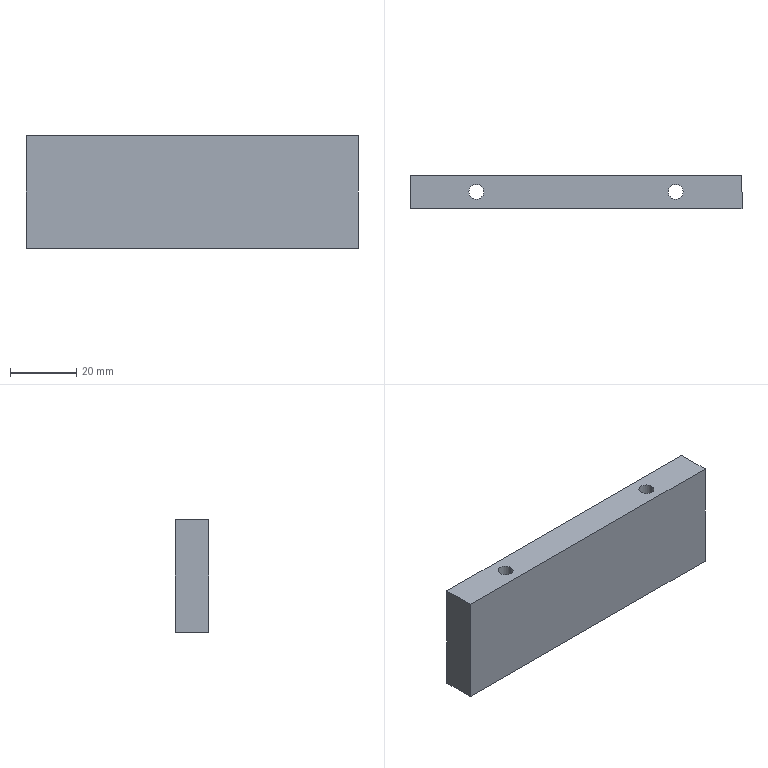Component | SolidWorks | 07-1111-1 | 1 solid | 28 faces | box 100 x 10 x 34 mm | volume 30538 mm3 | cylinder 14 | plane 8 | cone 6 | commonest cylinder face diameters 3.3 x6 8 x4 4.5 x4 | material AL6061(GB)Natural Anodized
build123d program:
from build123d import *

# Parameters (mm, degrees)
SKETCH1_W                                       = 100
SKETCH1_H                                       = 10
EXTRUDE1_DEPTH                                  = 34
M4_HEX_SOCKET_HEAD_CAP_SCREW_CBORE1_D           = 4.5
M4_HEX_SOCKET_HEAD_CAP_SCREW_CBORE1_CBORE_D     = 8
M4_HEX_SOCKET_HEAD_CAP_SCREW_CBORE1_CBORE_DEPTH = 30
M4_TAPPED_HOLE1_D                               = 3.3
M4_TAPPED_HOLE1_DEPTH                           = 12.1
M4_TAPPED_HOLE1_TIP                             = 0.9914


with BuildPart() as part:
    # Sketch1 → Extrude1 (new body)
    with BuildSketch(Plane.XY):
        with Locations((50, 5)):
            Rectangle(SKETCH1_W, SKETCH1_H)
    extrude(amount=EXTRUDE1_DEPTH)

    # M4 Hex Socket Head Cap Screw CBORE1 (through all)
    with Locations(Plane.XY.offset(34)):
        with Locations((20, 5), (80, 5)):
            CounterBoreHole(M4_HEX_SOCKET_HEAD_CAP_SCREW_CBORE1_D / 2, M4_HEX_SOCKET_HEAD_CAP_SCREW_CBORE1_CBORE_D / 2, M4_HEX_SOCKET_HEAD_CAP_SCREW_CBORE1_CBORE_DEPTH)

    # M4 Tapped Hole1
    with Locations(Plane.XY.offset(34)):
        with Locations((8, 5), (50, 5), (92, 5)):
            Hole(M4_TAPPED_HOLE1_D / 2, depth=M4_TAPPED_HOLE1_DEPTH)
            with Locations((0, 0, -(M4_TAPPED_HOLE1_DEPTH + M4_TAPPED_HOLE1_TIP / 2))):  # 118° drill point
                Cone(0, M4_TAPPED_HOLE1_D / 2, M4_TAPPED_HOLE1_TIP, mode=Mode.SUBTRACT)


solid = part.part

# Placed as in the assembly
solid = solid.moved(Location((-64.57, 60, -32), (180, 0, 0)))
STEP:
#1=CARTESIAN_POINT('',(-2.292,2.165,-2.122));
#2=VERTEX_POINT('',#1);
#3=CARTESIAN_POINT('',(-2.162,2.165,-2.122));
#4=VERTEX_POINT('',#3);
#5=CARTESIAN_POINT('',(-2.227,2.165,-2.122));
#6=DIRECTION('',(0.,0.,-1.));
#7=DIRECTION('',(1.,0.,0.));
#8=AXIS2_PLACEMENT_3D('',#5,#6,#7);
#9=CIRCLE('',#8,0.06496);
#10=EDGE_CURVE('',#2,#4,#9,.T.);
#11=ORIENTED_EDGE('',*,*,#10,.F.);
#12=CARTESIAN_POINT('',(-2.292,2.165,-2.598));
#13=VERTEX_POINT('',#12);
#14=CARTESIAN_POINT('',(-2.292,2.165,-2.598));
#15=DIRECTION('',(0.,0.,-1.));
#16=VECTOR('',#15,39.37);
#17=LINE('',#14,#16);
#18=EDGE_CURVE('',#2,#13,#17,.T.);
#19=ORIENTED_EDGE('',*,*,#18,.T.);
#20=CARTESIAN_POINT('',(-2.162,2.165,-2.598));
#21=VERTEX_POINT('',#20);
#22=CARTESIAN_POINT('',(-2.227,2.165,-2.598));
#23=DIRECTION('',(0.,0.,-1.));
#24=DIRECTION('',(1.,0.,0.));
#25=AXIS2_PLACEMENT_3D('',#22,#23,#24);
#26=CIRCLE('',#25,0.06496);
#27=EDGE_CURVE('',#13,#21,#26,.T.);
#28=ORIENTED_EDGE('',*,*,#27,.T.);
#29=CARTESIAN_POINT('',(-2.162,2.165,-2.598));
#30=DIRECTION('',(0.,0.,-1.));
#31=VECTOR('',#30,39.37);
#32=LINE('',#29,#31);
#33=EDGE_CURVE('',#4,#21,#32,.T.);
#34=ORIENTED_EDGE('',*,*,#33,.F.);
#35=EDGE_LOOP('',(#11,#19,#28,#34));
#36=FACE_OUTER_BOUND('',#35,.T.);
#37=CARTESIAN_POINT('',(-2.227,2.165,-2.598));
#38=DIRECTION('',(0.,0.,-1.));
#39=DIRECTION('',(1.,0.,0.));
#40=AXIS2_PLACEMENT_3D('',#37,#38,#39);
#41=CYLINDRICAL_SURFACE('',#40,0.06496);
#42=ADVANCED_FACE('',(#36),#41,.F.);
#43=CARTESIAN_POINT('',(-2.227,2.165,-2.083));
#44=VERTEX_POINT('',#43);
#45=CARTESIAN_POINT('',(-2.162,2.165,-2.122));
#46=DIRECTION('',(0.8572,0.,-0.515));
#47=VECTOR('',#46,39.37);
#48=LINE('',#45,#47);
#49=EDGE_CURVE('',#44,#4,#48,.T.);
#50=ORIENTED_EDGE('',*,*,#49,.F.);
#51=CARTESIAN_POINT('',(-2.292,2.165,-2.122));
#52=DIRECTION('',(-0.8572,-0.,-0.515));
#53=VECTOR('',#52,39.37);
#54=LINE('',#51,#53);
#55=EDGE_CURVE('',#44,#2,#54,.T.);
#56=ORIENTED_EDGE('',*,*,#55,.T.);
#57=ORIENTED_EDGE('',*,*,#10,.T.);
#58=EDGE_LOOP('',(#50,#56,#57));
#59=FACE_OUTER_BOUND('',#58,.T.);
#60=CARTESIAN_POINT('',(-2.227,2.165,-2.122));
#61=DIRECTION('',(0.,0.,-1.));
#62=DIRECTION('',(1.,0.,0.));
#63=AXIS2_PLACEMENT_3D('',#60,#61,#62);
#64=CONICAL_SURFACE('',#63,0.06496,1.03);
#65=ADVANCED_FACE('',(#59),#64,.F.);
#66=CARTESIAN_POINT('',(-0.6386,2.165,-2.122));
#67=VERTEX_POINT('',#66);
#68=CARTESIAN_POINT('',(-0.5087,2.165,-2.122));
#69=VERTEX_POINT('',#68);
#70=CARTESIAN_POINT('',(-0.5736,2.165,-2.122));
#71=DIRECTION('',(0.,0.,-1.));
#72=DIRECTION('',(1.,0.,0.));
#73=AXIS2_PLACEMENT_3D('',#70,#71,#72);
#74=CIRCLE('',#73,0.06496);
#75=EDGE_CURVE('',#67,#69,#74,.T.);
#76=ORIENTED_EDGE('',*,*,#75,.F.);
#77=CARTESIAN_POINT('',(-0.6386,2.165,-2.598));
#78=VERTEX_POINT('',#77);
#79=CARTESIAN_POINT('',(-0.6386,2.165,-2.598));
#80=DIRECTION('',(0.,0.,-1.));
#81=VECTOR('',#80,39.37);
#82=LINE('',#79,#81);
#83=EDGE_CURVE('',#67,#78,#82,.T.);
#84=ORIENTED_EDGE('',*,*,#83,.T.);
#85=CARTESIAN_POINT('',(-0.5087,2.165,-2.598));
#86=VERTEX_POINT('',#85);
#87=CARTESIAN_POINT('',(-0.5736,2.165,-2.598));
#88=DIRECTION('',(0.,0.,-1.));
#89=DIRECTION('',(1.,0.,0.));
#90=AXIS2_PLACEMENT_3D('',#87,#88,#89);
#91=CIRCLE('',#90,0.06496);
#92=EDGE_CURVE('',#78,#86,#91,.T.);
#93=ORIENTED_EDGE('',*,*,#92,.T.);
#94=CARTESIAN_POINT('',(-0.5087,2.165,-2.598));
#95=DIRECTION('',(0.,0.,-1.));
#96=VECTOR('',#95,39.37);
#97=LINE('',#94,#96);
#98=EDGE_CURVE('',#69,#86,#97,.T.);
#99=ORIENTED_EDGE('',*,*,#98,.F.);
#100=EDGE_LOOP('',(#76,#84,#93,#99));
#101=FACE_OUTER_BOUND('',#100,.T.);
#102=CARTESIAN_POINT('',(-0.5736,2.165,-2.598));
#103=DIRECTION('',(0.,0.,-1.));
#104=DIRECTION('',(1.,0.,0.));
#105=AXIS2_PLACEMENT_3D('',#102,#103,#104);
#106=CYLINDRICAL_SURFACE('',#105,0.06496);
#107=ADVANCED_FACE('',(#101),#106,.F.);
#108=CARTESIAN_POINT('',(-0.5736,2.165,-2.083));
#109=VERTEX_POINT('',#108);
#110=CARTESIAN_POINT('',(-0.5087,2.165,-2.122));
#111=DIRECTION('',(0.8572,0.,-0.515));
#112=VECTOR('',#111,39.37);
#113=LINE('',#110,#112);
#114=EDGE_CURVE('',#109,#69,#113,.T.);
#115=ORIENTED_EDGE('',*,*,#114,.F.);
#116=CARTESIAN_POINT('',(-0.6386,2.165,-2.122));
#117=DIRECTION('',(-0.8572,-0.,-0.515));
#118=VECTOR('',#117,39.37);
#119=LINE('',#116,#118);
#120=EDGE_CURVE('',#109,#67,#119,.T.);
#121=ORIENTED_EDGE('',*,*,#120,.T.);
#122=ORIENTED_EDGE('',*,*,#75,.T.);
#123=EDGE_LOOP('',(#115,#121,#122));
#124=FACE_OUTER_BOUND('',#123,.T.);
#125=CARTESIAN_POINT('',(-0.5736,2.165,-2.122));
#126=DIRECTION('',(0.,0.,-1.));
#127=DIRECTION('',(1.,0.,0.));
#128=AXIS2_PLACEMENT_3D('',#125,#126,#127);
#129=CONICAL_SURFACE('',#128,0.06496,1.03);
#130=ADVANCED_FACE('',(#124),#129,.F.);
#131=CARTESIAN_POINT('',(1.015,2.165,-2.122));
#132=VERTEX_POINT('',#131);
#133=CARTESIAN_POINT('',(1.145,2.165,-2.122));
#134=VERTEX_POINT('',#133);
#135=CARTESIAN_POINT('',(1.08,2.165,-2.122));
#136=DIRECTION('',(0.,0.,-1.));
#137=DIRECTION('',(1.,0.,0.));
#138=AXIS2_PLACEMENT_3D('',#135,#136,#137);
#139=CIRCLE('',#138,0.06496);
#140=EDGE_CURVE('',#132,#134,#139,.T.);
#141=ORIENTED_EDGE('',*,*,#140,.F.);
#142=CARTESIAN_POINT('',(1.015,2.165,-2.598));
#143=VERTEX_POINT('',#142);
#144=CARTESIAN_POINT('',(1.015,2.165,-2.598));
#145=DIRECTION('',(0.,0.,-1.));
#146=VECTOR('',#145,39.37);
#147=LINE('',#144,#146);
#148=EDGE_CURVE('',#132,#143,#147,.T.);
#149=ORIENTED_EDGE('',*,*,#148,.T.);
#150=CARTESIAN_POINT('',(1.145,2.165,-2.598));
#151=VERTEX_POINT('',#150);
#152=CARTESIAN_POINT('',(1.08,2.165,-2.598));
#153=DIRECTION('',(0.,0.,-1.));
#154=DIRECTION('',(1.,0.,0.));
#155=AXIS2_PLACEMENT_3D('',#152,#153,#154);
#156=CIRCLE('',#155,0.06496);
#157=EDGE_CURVE('',#143,#151,#156,.T.);
#158=ORIENTED_EDGE('',*,*,#157,.T.);
#159=CARTESIAN_POINT('',(1.145,2.165,-2.598));
#160=DIRECTION('',(0.,0.,-1.));
#161=VECTOR('',#160,39.37);
#162=LINE('',#159,#161);
#163=EDGE_CURVE('',#134,#151,#162,.T.);
#164=ORIENTED_EDGE('',*,*,#163,.F.);
#165=EDGE_LOOP('',(#141,#149,#158,#164));
#166=FACE_OUTER_BOUND('',#165,.T.);
#167=CARTESIAN_POINT('',(1.08,2.165,-2.598));
#168=DIRECTION('',(0.,0.,-1.));
#169=DIRECTION('',(1.,0.,0.));
#170=AXIS2_PLACEMENT_3D('',#167,#168,#169);
#171=CYLINDRICAL_SURFACE('',#170,0.06496);
#172=ADVANCED_FACE('',(#166),#171,.F.);
#173=CARTESIAN_POINT('',(1.08,2.165,-2.083));
#174=VERTEX_POINT('',#173);
#175=CARTESIAN_POINT('',(1.145,2.165,-2.122));
#176=DIRECTION('',(0.8572,0.,-0.515));
#177=VECTOR('',#176,39.37);
#178=LINE('',#175,#177);
#179=EDGE_CURVE('',#174,#134,#178,.T.);
#180=ORIENTED_EDGE('',*,*,#179,.F.);
#181=CARTESIAN_POINT('',(1.015,2.165,-2.122));
#182=DIRECTION('',(-0.8572,-0.,-0.515));
#183=VECTOR('',#182,39.37);
#184=LINE('',#181,#183);
#185=EDGE_CURVE('',#174,#132,#184,.T.);
#186=ORIENTED_EDGE('',*,*,#185,.T.);
#187=ORIENTED_EDGE('',*,*,#140,.T.);
#188=EDGE_LOOP('',(#180,#186,#187));
#189=FACE_OUTER_BOUND('',#188,.T.);
#190=CARTESIAN_POINT('',(1.08,2.165,-2.122));
#191=DIRECTION('',(0.,0.,-1.));
#192=DIRECTION('',(1.,0.,0.));
#193=AXIS2_PLACEMENT_3D('',#190,#191,#192);
#194=CONICAL_SURFACE('',#193,0.06496,1.03);
#195=ADVANCED_FACE('',(#189),#194,.F.);
#196=CARTESIAN_POINT('',(-1.912,2.165,-1.417));
#197=VERTEX_POINT('',#196);
#198=CARTESIAN_POINT('',(-1.597,2.165,-1.417));
#199=VERTEX_POINT('',#198);
#200=CARTESIAN_POINT('',(-1.755,2.165,-1.417));
#201=DIRECTION('',(0.,0.,-1.));
#202=DIRECTION('',(1.,0.,0.));
#203=AXIS2_PLACEMENT_3D('',#200,#201,#202);
#204=CIRCLE('',#203,0.1575);
#205=EDGE_CURVE('',#197,#199,#204,.T.);
#206=ORIENTED_EDGE('',*,*,#205,.F.);
#207=CARTESIAN_POINT('',(-1.912,2.165,-2.598));
#208=VERTEX_POINT('',#207);
#209=CARTESIAN_POINT('',(-1.912,2.165,-2.598));
#210=DIRECTION('',(0.,0.,-1.));
#211=VECTOR('',#210,39.37);
#212=LINE('',#209,#211);
#213=EDGE_CURVE('',#197,#208,#212,.T.);
#214=ORIENTED_EDGE('',*,*,#213,.T.);
#215=CARTESIAN_POINT('',(-1.597,2.165,-2.598));
#216=VERTEX_POINT('',#215);
#217=CARTESIAN_POINT('',(-1.755,2.165,-2.598));
#218=DIRECTION('',(0.,0.,-1.));
#219=DIRECTION('',(1.,0.,0.));
#220=AXIS2_PLACEMENT_3D('',#217,#218,#219);
#221=CIRCLE('',#220,0.1575);
#222=EDGE_CURVE('',#208,#216,#221,.T.);
#223=ORIENTED_EDGE('',*,*,#222,.T.);
#224=CARTESIAN_POINT('',(-1.597,2.165,-2.598));
#225=DIRECTION('',(0.,0.,-1.));
#226=VECTOR('',#225,39.37);
#227=LINE('',#224,#226);
#228=EDGE_CURVE('',#199,#216,#227,.T.);
#229=ORIENTED_EDGE('',*,*,#228,.F.);
#230=EDGE_LOOP('',(#206,#214,#223,#229));
#231=FACE_OUTER_BOUND('',#230,.T.);
#232=CARTESIAN_POINT('',(-1.755,2.165,-2.598));
#233=DIRECTION('',(0.,0.,-1.));
#234=DIRECTION('',(1.,0.,0.));
#235=AXIS2_PLACEMENT_3D('',#232,#233,#234);
#236=CYLINDRICAL_SURFACE('',#235,0.1575);
#237=ADVANCED_FACE('',(#231),#236,.F.);
#238=CARTESIAN_POINT('',(-1.843,2.165,-1.26));
#239=VERTEX_POINT('',#238);
#240=CARTESIAN_POINT('',(-1.666,2.165,-1.26));
#241=VERTEX_POINT('',#240);
#242=CARTESIAN_POINT('',(-1.755,2.165,-1.26));
#243=DIRECTION('',(0.,0.,-1.));
#244=DIRECTION('',(1.,0.,0.));
#245=AXIS2_PLACEMENT_3D('',#242,#243,#244);
#246=CIRCLE('',#245,0.08858);
#247=EDGE_CURVE('',#239,#241,#246,.T.);
#248=ORIENTED_EDGE('',*,*,#247,.F.);
#249=CARTESIAN_POINT('',(-1.843,2.165,-1.417));
#250=VERTEX_POINT('',#249);
#251=CARTESIAN_POINT('',(-1.843,2.165,-2.598));
#252=DIRECTION('',(0.,0.,-1.));
#253=VECTOR('',#252,39.37);
#254=LINE('',#251,#253);
#255=EDGE_CURVE('',#239,#250,#254,.T.);
#256=ORIENTED_EDGE('',*,*,#255,.T.);
#257=CARTESIAN_POINT('',(-1.666,2.165,-1.417));
#258=VERTEX_POINT('',#257);
#259=CARTESIAN_POINT('',(-1.755,2.165,-1.417));
#260=DIRECTION('',(0.,0.,-1.));
#261=DIRECTION('',(1.,0.,0.));
#262=AXIS2_PLACEMENT_3D('',#259,#260,#261);
#263=CIRCLE('',#262,0.08858);
#264=EDGE_CURVE('',#250,#258,#263,.T.);
#265=ORIENTED_EDGE('',*,*,#264,.T.);
#266=CARTESIAN_POINT('',(-1.666,2.165,-2.598));
#267=DIRECTION('',(0.,0.,-1.));
#268=VECTOR('',#267,39.37);
#269=LINE('',#266,#268);
#270=EDGE_CURVE('',#241,#258,#269,.T.);
#271=ORIENTED_EDGE('',*,*,#270,.F.);
#272=EDGE_LOOP('',(#248,#256,#265,#271));
#273=FACE_OUTER_BOUND('',#272,.T.);
#274=CARTESIAN_POINT('',(-1.755,2.165,-2.598));
#275=DIRECTION('',(0.,0.,-1.));
#276=DIRECTION('',(1.,0.,0.));
#277=AXIS2_PLACEMENT_3D('',#274,#275,#276);
#278=CYLINDRICAL_SURFACE('',#277,0.08858);
#279=ADVANCED_FACE('',(#273),#278,.F.);
#280=CARTESIAN_POINT('',(0.45,2.165,-1.417));
#281=VERTEX_POINT('',#280);
#282=CARTESIAN_POINT('',(0.765,2.165,-1.417));
#283=VERTEX_POINT('',#282);
#284=CARTESIAN_POINT('',(0.6075,2.165,-1.417));
#285=DIRECTION('',(0.,0.,-1.));
#286=DIRECTION('',(1.,0.,0.));
#287=AXIS2_PLACEMENT_3D('',#284,#285,#286);
#288=CIRCLE('',#287,0.1575);
#289=EDGE_CURVE('',#281,#283,#288,.T.);
#290=ORIENTED_EDGE('',*,*,#289,.F.);
#291=CARTESIAN_POINT('',(0.45,2.165,-2.598));
#292=VERTEX_POINT('',#291);
#293=CARTESIAN_POINT('',(0.45,2.165,-2.598));
#294=DIRECTION('',(0.,0.,-1.));
#295=VECTOR('',#294,39.37);
#296=LINE('',#293,#295);
#297=EDGE_CURVE('',#281,#292,#296,.T.);
#298=ORIENTED_EDGE('',*,*,#297,.T.);
#299=CARTESIAN_POINT('',(0.765,2.165,-2.598));
#300=VERTEX_POINT('',#299);
#301=CARTESIAN_POINT('',(0.6075,2.165,-2.598));
#302=DIRECTION('',(0.,0.,-1.));
#303=DIRECTION('',(1.,0.,0.));
#304=AXIS2_PLACEMENT_3D('',#301,#302,#303);
#305=CIRCLE('',#304,0.1575);
#306=EDGE_CURVE('',#292,#300,#305,.T.);
#307=ORIENTED_EDGE('',*,*,#306,.T.);
#308=CARTESIAN_POINT('',(0.765,2.165,-2.598));
#309=DIRECTION('',(0.,0.,-1.));
#310=VECTOR('',#309,39.37);
#311=LINE('',#308,#310);
#312=EDGE_CURVE('',#283,#300,#311,.T.);
#313=ORIENTED_EDGE('',*,*,#312,.F.);
#314=EDGE_LOOP('',(#290,#298,#307,#313));
#315=FACE_OUTER_BOUND('',#314,.T.);
#316=CARTESIAN_POINT('',(0.6075,2.165,-2.598));
#317=DIRECTION('',(0.,0.,-1.));
#318=DIRECTION('',(1.,0.,0.));
#319=AXIS2_PLACEMENT_3D('',#316,#317,#318);
#320=CYLINDRICAL_SURFACE('',#319,0.1575);
#321=ADVANCED_FACE('',(#315),#320,.F.);
#322=CARTESIAN_POINT('',(0.5189,2.165,-1.26));
#323=VERTEX_POINT('',#322);
#324=CARTESIAN_POINT('',(0.6961,2.165,-1.26));
#325=VERTEX_POINT('',#324);
#326=CARTESIAN_POINT('',(0.6075,2.165,-1.26));
#327=DIRECTION('',(0.,0.,-1.));
#328=DIRECTION('',(1.,0.,0.));
#329=AXIS2_PLACEMENT_3D('',#326,#327,#328);
#330=CIRCLE('',#329,0.08858);
#331=EDGE_CURVE('',#323,#325,#330,.T.);
#332=ORIENTED_EDGE('',*,*,#331,.F.);
#333=CARTESIAN_POINT('',(0.5189,2.165,-1.417));
#334=VERTEX_POINT('',#333);
#335=CARTESIAN_POINT('',(0.5189,2.165,-2.598));
#336=DIRECTION('',(0.,0.,-1.));
#337=VECTOR('',#336,39.37);
#338=LINE('',#335,#337);
#339=EDGE_CURVE('',#323,#334,#338,.T.);
#340=ORIENTED_EDGE('',*,*,#339,.T.);
#341=CARTESIAN_POINT('',(0.6961,2.165,-1.417));
#342=VERTEX_POINT('',#341);
#343=CARTESIAN_POINT('',(0.6075,2.165,-1.417));
#344=DIRECTION('',(0.,0.,-1.));
#345=DIRECTION('',(1.,0.,0.));
#346=AXIS2_PLACEMENT_3D('',#343,#344,#345);
#347=CIRCLE('',#346,0.08858);
#348=EDGE_CURVE('',#334,#342,#347,.T.);
#349=ORIENTED_EDGE('',*,*,#348,.T.);
#350=CARTESIAN_POINT('',(0.6961,2.165,-2.598));
#351=DIRECTION('',(0.,0.,-1.));
#352=VECTOR('',#351,39.37);
#353=LINE('',#350,#352);
#354=EDGE_CURVE('',#325,#342,#353,.T.);
#355=ORIENTED_EDGE('',*,*,#354,.F.);
#356=EDGE_LOOP('',(#332,#340,#349,#355));
#357=FACE_OUTER_BOUND('',#356,.T.);
#358=CARTESIAN_POINT('',(0.6075,2.165,-2.598));
#359=DIRECTION('',(0.,0.,-1.));
#360=DIRECTION('',(1.,0.,0.));
#361=AXIS2_PLACEMENT_3D('',#358,#359,#360);
#362=CYLINDRICAL_SURFACE('',#361,0.08858);
#363=ADVANCED_FACE('',(#357),#362,.F.);
#364=CARTESIAN_POINT('',(-2.542,1.969,-1.26));
#365=VERTEX_POINT('',#364);
#366=CARTESIAN_POINT('',(-2.542,2.362,-1.26));
#367=VERTEX_POINT('',#366);
#368=CARTESIAN_POINT('',(-2.542,2.362,-1.26));
#369=DIRECTION('',(-0.,1.,-0.));
#370=VECTOR('',#369,39.37);
#371=LINE('',#368,#370);
#372=EDGE_CURVE('',#365,#367,#371,.T.);
#373=ORIENTED_EDGE('',*,*,#372,.T.);
#374=CARTESIAN_POINT('',(-2.542,2.362,-2.598));
#375=VERTEX_POINT('',#374);
#376=CARTESIAN_POINT('',(-2.542,2.362,-2.598));
#377=DIRECTION('',(-0.,-0.,1.));
#378=VECTOR('',#377,39.37);
#379=LINE('',#376,#378);
#380=EDGE_CURVE('',#375,#367,#379,.T.);
#381=ORIENTED_EDGE('',*,*,#380,.F.);
#382=CARTESIAN_POINT('',(-2.542,1.969,-2.598));
#383=VERTEX_POINT('',#382);
#384=CARTESIAN_POINT('',(-2.542,2.362,-2.598));
#385=DIRECTION('',(-0.,1.,-0.));
#386=VECTOR('',#385,39.37);
#387=LINE('',#384,#386);
#388=EDGE_CURVE('',#383,#375,#387,.T.);
#389=ORIENTED_EDGE('',*,*,#388,.F.);
#390=CARTESIAN_POINT('',(-2.542,1.969,-2.598));
#391=DIRECTION('',(-0.,-0.,1.));
#392=VECTOR('',#391,39.37);
#393=LINE('',#390,#392);
#394=EDGE_CURVE('',#383,#365,#393,.T.);
#395=ORIENTED_EDGE('',*,*,#394,.T.);
#396=EDGE_LOOP('',(#373,#381,#389,#395));
#397=FACE_OUTER_BOUND('',#396,.T.);
#398=CARTESIAN_POINT('',(-2.542,2.362,-2.598));
#399=DIRECTION('',(1.,0.,0.));
#400=DIRECTION('',(-0.,-0.,1.));
#401=AXIS2_PLACEMENT_3D('',#398,#399,#400);
#402=PLANE('',#401);
#403=ADVANCED_FACE('',(#397),#402,.F.);
#404=CARTESIAN_POINT('',(1.395,2.362,-1.26));
#405=VERTEX_POINT('',#404);
#406=CARTESIAN_POINT('',(-2.542,2.362,-1.26));
#407=DIRECTION('',(1.,0.,0.));
#408=VECTOR('',#407,39.37);
#409=LINE('',#406,#408);
#410=EDGE_CURVE('',#367,#405,#409,.T.);
#411=ORIENTED_EDGE('',*,*,#410,.T.);
#412=CARTESIAN_POINT('',(1.395,2.362,-2.598));
#413=VERTEX_POINT('',#412);
#414=CARTESIAN_POINT('',(1.395,2.362,-2.598));
#415=DIRECTION('',(-0.,-0.,1.));
#416=VECTOR('',#415,39.37);
#417=LINE('',#414,#416);
#418=EDGE_CURVE('',#413,#405,#417,.T.);
#419=ORIENTED_EDGE('',*,*,#418,.F.);
#420=CARTESIAN_POINT('',(-2.542,2.362,-2.598));
#421=DIRECTION('',(1.,0.,0.));
#422=VECTOR('',#421,39.37);
#423=LINE('',#420,#422);
#424=EDGE_CURVE('',#375,#413,#423,.T.);
#425=ORIENTED_EDGE('',*,*,#424,.F.);
#426=ORIENTED_EDGE('',*,*,#380,.T.);
#427=EDGE_LOOP('',(#411,#419,#425,#426));
#428=FACE_OUTER_BOUND('',#427,.T.);
#429=CARTESIAN_POINT('',(-2.542,2.362,-2.598));
#430=DIRECTION('',(0.,-1.,-0.));
#431=DIRECTION('',(0.,0.,-1.));
#432=AXIS2_PLACEMENT_3D('',#429,#430,#431);
#433=PLANE('',#432);
#434=ADVANCED_FACE('',(#428),#433,.F.);
#435=CARTESIAN_POINT('',(1.395,1.969,-1.26));
#436=VERTEX_POINT('',#435);
#437=CARTESIAN_POINT('',(1.395,2.362,-1.26));
#438=DIRECTION('',(0.,-1.,0.));
#439=VECTOR('',#438,39.37);
#440=LINE('',#437,#439);
#441=EDGE_CURVE('',#405,#436,#440,.T.);
#442=ORIENTED_EDGE('',*,*,#441,.T.);
#443=CARTESIAN_POINT('',(1.395,1.969,-2.598));
#444=VERTEX_POINT('',#443);
#445=CARTESIAN_POINT('',(1.395,1.969,-2.598));
#446=DIRECTION('',(-0.,-0.,1.));
#447=VECTOR('',#446,39.37);
#448=LINE('',#445,#447);
#449=EDGE_CURVE('',#444,#436,#448,.T.);
#450=ORIENTED_EDGE('',*,*,#449,.F.);
#451=CARTESIAN_POINT('',(1.395,2.362,-2.598));
#452=DIRECTION('',(0.,-1.,0.));
#453=VECTOR('',#452,39.37);
#454=LINE('',#451,#453);
#455=EDGE_CURVE('',#413,#444,#454,.T.);
#456=ORIENTED_EDGE('',*,*,#455,.F.);
#457=ORIENTED_EDGE('',*,*,#418,.T.);
#458=EDGE_LOOP('',(#442,#450,#456,#457));
#459=FACE_OUTER_BOUND('',#458,.T.);
#460=CARTESIAN_POINT('',(1.395,2.362,-2.598));
#461=DIRECTION('',(-1.,-0.,-0.));
#462=DIRECTION('',(0.,0.,-1.));
#463=AXIS2_PLACEMENT_3D('',#460,#461,#462);
#464=PLANE('',#463);
#465=ADVANCED_FACE('',(#459),#464,.F.);
#466=CARTESIAN_POINT('',(-2.542,1.969,-1.26));
#467=DIRECTION('',(-1.,-0.,-0.));
#468=VECTOR('',#467,39.37);
#469=LINE('',#466,#468);
#470=EDGE_CURVE('',#436,#365,#469,.T.);
#471=ORIENTED_EDGE('',*,*,#470,.T.);
#472=ORIENTED_EDGE('',*,*,#394,.F.);
#473=CARTESIAN_POINT('',(-2.542,1.969,-2.598));
#474=DIRECTION('',(-1.,-0.,-0.));
#475=VECTOR('',#474,39.37);
#476=LINE('',#473,#475);
#477=EDGE_CURVE('',#444,#383,#476,.T.);
#478=ORIENTED_EDGE('',*,*,#477,.F.);
#479=ORIENTED_EDGE('',*,*,#449,.T.);
#480=EDGE_LOOP('',(#471,#472,#478,#479));
#481=FACE_OUTER_BOUND('',#480,.T.);
#482=CARTESIAN_POINT('',(-2.542,1.969,-2.598));
#483=DIRECTION('',(-0.,1.,0.));
#484=DIRECTION('',(-0.,-0.,1.));
#485=AXIS2_PLACEMENT_3D('',#482,#483,#484);
#486=PLANE('',#485);
#487=ADVANCED_FACE('',(#481),#486,.F.);
#488=CARTESIAN_POINT('',(-2.227,2.165,-2.598));
#489=DIRECTION('',(0.,0.,-1.));
#490=DIRECTION('',(1.,0.,0.));
#491=AXIS2_PLACEMENT_3D('',#488,#489,#490);
#492=CIRCLE('',#491,0.06496);
#493=EDGE_CURVE('',#21,#13,#492,.T.);
#494=ORIENTED_EDGE('',*,*,#493,.F.);
#495=ORIENTED_EDGE('',*,*,#27,.F.);
#496=EDGE_LOOP('',(#494,#495));
#497=FACE_BOUND('',#496,.T.);
#498=CARTESIAN_POINT('',(-0.5736,2.165,-2.598));
#499=DIRECTION('',(0.,0.,-1.));
#500=DIRECTION('',(1.,0.,0.));
#501=AXIS2_PLACEMENT_3D('',#498,#499,#500);
#502=CIRCLE('',#501,0.06496);
#503=EDGE_CURVE('',#86,#78,#502,.T.);
#504=ORIENTED_EDGE('',*,*,#503,.F.);
#505=ORIENTED_EDGE('',*,*,#92,.F.);
#506=EDGE_LOOP('',(#504,#505));
#507=FACE_BOUND('',#506,.T.);
#508=CARTESIAN_POINT('',(1.08,2.165,-2.598));
#509=DIRECTION('',(0.,0.,-1.));
#510=DIRECTION('',(1.,0.,0.));
#511=AXIS2_PLACEMENT_3D('',#508,#509,#510);
#512=CIRCLE('',#511,0.06496);
#513=EDGE_CURVE('',#151,#143,#512,.T.);
#514=ORIENTED_EDGE('',*,*,#513,.F.);
#515=ORIENTED_EDGE('',*,*,#157,.F.);
#516=EDGE_LOOP('',(#514,#515));
#517=FACE_BOUND('',#516,.T.);
#518=CARTESIAN_POINT('',(-1.755,2.165,-2.598));
#519=DIRECTION('',(0.,0.,-1.));
#520=DIRECTION('',(1.,0.,0.));
#521=AXIS2_PLACEMENT_3D('',#518,#519,#520);
#522=CIRCLE('',#521,0.1575);
#523=EDGE_CURVE('',#216,#208,#522,.T.);
#524=ORIENTED_EDGE('',*,*,#523,.F.);
#525=ORIENTED_EDGE('',*,*,#222,.F.);
#526=EDGE_LOOP('',(#524,#525));
#527=FACE_BOUND('',#526,.T.);
#528=CARTESIAN_POINT('',(0.6075,2.165,-2.598));
#529=DIRECTION('',(0.,0.,-1.));
#530=DIRECTION('',(1.,0.,0.));
#531=AXIS2_PLACEMENT_3D('',#528,#529,#530);
#532=CIRCLE('',#531,0.1575);
#533=EDGE_CURVE('',#300,#292,#532,.T.);
#534=ORIENTED_EDGE('',*,*,#533,.F.);
#535=ORIENTED_EDGE('',*,*,#306,.F.);
#536=EDGE_LOOP('',(#534,#535));
#537=FACE_BOUND('',#536,.T.);
#538=ORIENTED_EDGE('',*,*,#388,.T.);
#539=ORIENTED_EDGE('',*,*,#424,.T.);
#540=ORIENTED_EDGE('',*,*,#455,.T.);
#541=ORIENTED_EDGE('',*,*,#477,.T.);
#542=EDGE_LOOP('',(#538,#539,#540,#541));
#543=FACE_OUTER_BOUND('',#542,.T.);
#544=CARTESIAN_POINT('',(-2.542,1.969,-2.598));
#545=DIRECTION('',(-0.,-0.,1.));
#546=DIRECTION('',(-1.,-0.,-0.));
#547=AXIS2_PLACEMENT_3D('',#544,#545,#546);
#548=PLANE('',#547);
#549=ADVANCED_FACE('',(#497,#507,#517,#527,#537,#543),#548,.F.);
#550=CARTESIAN_POINT('',(-1.755,2.165,-1.26));
#551=DIRECTION('',(0.,0.,-1.));
#552=DIRECTION('',(1.,0.,0.));
#553=AXIS2_PLACEMENT_3D('',#550,#551,#552);
#554=CIRCLE('',#553,0.08858);
#555=EDGE_CURVE('',#241,#239,#554,.T.);
#556=ORIENTED_EDGE('',*,*,#555,.T.);
#557=ORIENTED_EDGE('',*,*,#247,.T.);
#558=EDGE_LOOP('',(#556,#557));
#559=FACE_BOUND('',#558,.T.);
#560=CARTESIAN_POINT('',(0.6075,2.165,-1.26));
#561=DIRECTION('',(0.,0.,-1.));
#562=DIRECTION('',(1.,0.,0.));
#563=AXIS2_PLACEMENT_3D('',#560,#561,#562);
#564=CIRCLE('',#563,0.08858);
#565=EDGE_CURVE('',#325,#323,#564,.T.);
#566=ORIENTED_EDGE('',*,*,#565,.T.);
#567=ORIENTED_EDGE('',*,*,#331,.T.);
#568=EDGE_LOOP('',(#566,#567));
#569=FACE_BOUND('',#568,.T.);
#570=ORIENTED_EDGE('',*,*,#372,.F.);
#571=ORIENTED_EDGE('',*,*,#470,.F.);
#572=ORIENTED_EDGE('',*,*,#441,.F.);
#573=ORIENTED_EDGE('',*,*,#410,.F.);
#574=EDGE_LOOP('',(#570,#571,#572,#573));
#575=FACE_OUTER_BOUND('',#574,.T.);
#576=CARTESIAN_POINT('',(-2.542,1.969,-1.26));
#577=DIRECTION('',(-0.,-0.,1.));
#578=DIRECTION('',(-1.,-0.,-0.));
#579=AXIS2_PLACEMENT_3D('',#576,#577,#578);
#580=PLANE('',#579);
#581=ADVANCED_FACE('',(#559,#569,#575),#580,.T.);
#582=ORIENTED_EDGE('',*,*,#339,.F.);
#583=ORIENTED_EDGE('',*,*,#565,.F.);
#584=ORIENTED_EDGE('',*,*,#354,.T.);
#585=CARTESIAN_POINT('',(0.6075,2.165,-1.417));
#586=DIRECTION('',(0.,0.,-1.));
#587=DIRECTION('',(1.,0.,0.));
#588=AXIS2_PLACEMENT_3D('',#585,#586,#587);
#589=CIRCLE('',#588,0.08858);
#590=EDGE_CURVE('',#342,#334,#589,.T.);
#591=ORIENTED_EDGE('',*,*,#590,.T.);
#592=EDGE_LOOP('',(#582,#583,#584,#591));
#593=FACE_OUTER_BOUND('',#592,.T.);
#594=CARTESIAN_POINT('',(0.6075,2.165,-2.598));
#595=DIRECTION('',(0.,0.,-1.));
#596=DIRECTION('',(1.,0.,0.));
#597=AXIS2_PLACEMENT_3D('',#594,#595,#596);
#598=CYLINDRICAL_SURFACE('',#597,0.08858);
#599=ADVANCED_FACE('',(#593),#598,.F.);
#600=ORIENTED_EDGE('',*,*,#590,.F.);
#601=ORIENTED_EDGE('',*,*,#348,.F.);
#602=EDGE_LOOP('',(#600,#601));
#603=FACE_BOUND('',#602,.T.);
#604=CARTESIAN_POINT('',(0.6075,2.165,-1.417));
#605=DIRECTION('',(0.,0.,-1.));
#606=DIRECTION('',(1.,0.,0.));
#607=AXIS2_PLACEMENT_3D('',#604,#605,#606);
#608=CIRCLE('',#607,0.1575);
#609=EDGE_CURVE('',#283,#281,#608,.T.);
#610=ORIENTED_EDGE('',*,*,#609,.T.);
#611=ORIENTED_EDGE('',*,*,#289,.T.);
#612=EDGE_LOOP('',(#610,#611));
#613=FACE_OUTER_BOUND('',#612,.T.);
#614=CARTESIAN_POINT('',(0.6961,2.165,-1.417));
#615=DIRECTION('',(-0.,-0.,1.));
#616=DIRECTION('',(-1.,-0.,-0.));
#617=AXIS2_PLACEMENT_3D('',#614,#615,#616);
#618=PLANE('',#617);
#619=ADVANCED_FACE('',(#603,#613),#618,.F.);
#620=ORIENTED_EDGE('',*,*,#297,.F.);
#621=ORIENTED_EDGE('',*,*,#609,.F.);
#622=ORIENTED_EDGE('',*,*,#312,.T.);
#623=ORIENTED_EDGE('',*,*,#533,.T.);
#624=EDGE_LOOP('',(#620,#621,#622,#623));
#625=FACE_OUTER_BOUND('',#624,.T.);
#626=CARTESIAN_POINT('',(0.6075,2.165,-2.598));
#627=DIRECTION('',(0.,0.,-1.));
#628=DIRECTION('',(1.,0.,0.));
#629=AXIS2_PLACEMENT_3D('',#626,#627,#628);
#630=CYLINDRICAL_SURFACE('',#629,0.1575);
#631=ADVANCED_FACE('',(#625),#630,.F.);
#632=ORIENTED_EDGE('',*,*,#255,.F.);
#633=ORIENTED_EDGE('',*,*,#555,.F.);
#634=ORIENTED_EDGE('',*,*,#270,.T.);
#635=CARTESIAN_POINT('',(-1.755,2.165,-1.417));
#636=DIRECTION('',(0.,0.,-1.));
#637=DIRECTION('',(1.,0.,0.));
#638=AXIS2_PLACEMENT_3D('',#635,#636,#637);
#639=CIRCLE('',#638,0.08858);
#640=EDGE_CURVE('',#258,#250,#639,.T.);
#641=ORIENTED_EDGE('',*,*,#640,.T.);
#642=EDGE_LOOP('',(#632,#633,#634,#641));
#643=FACE_OUTER_BOUND('',#642,.T.);
#644=CARTESIAN_POINT('',(-1.755,2.165,-2.598));
#645=DIRECTION('',(0.,0.,-1.));
#646=DIRECTION('',(1.,0.,0.));
#647=AXIS2_PLACEMENT_3D('',#644,#645,#646);
#648=CYLINDRICAL_SURFACE('',#647,0.08858);
#649=ADVANCED_FACE('',(#643),#648,.F.);
#650=ORIENTED_EDGE('',*,*,#640,.F.);
#651=ORIENTED_EDGE('',*,*,#264,.F.);
#652=EDGE_LOOP('',(#650,#651));
#653=FACE_BOUND('',#652,.T.);
#654=CARTESIAN_POINT('',(-1.755,2.165,-1.417));
#655=DIRECTION('',(0.,0.,-1.));
#656=DIRECTION('',(1.,0.,0.));
#657=AXIS2_PLACEMENT_3D('',#654,#655,#656);
#658=CIRCLE('',#657,0.1575);
#659=EDGE_CURVE('',#199,#197,#658,.T.);
#660=ORIENTED_EDGE('',*,*,#659,.T.);
#661=ORIENTED_EDGE('',*,*,#205,.T.);
#662=EDGE_LOOP('',(#660,#661));
#663=FACE_OUTER_BOUND('',#662,.T.);
#664=CARTESIAN_POINT('',(-1.666,2.165,-1.417));
#665=DIRECTION('',(-0.,-0.,1.));
#666=DIRECTION('',(-1.,-0.,-0.));
#667=AXIS2_PLACEMENT_3D('',#664,#665,#666);
#668=PLANE('',#667);
#669=ADVANCED_FACE('',(#653,#663),#668,.F.);
#670=ORIENTED_EDGE('',*,*,#213,.F.);
#671=ORIENTED_EDGE('',*,*,#659,.F.);
#672=ORIENTED_EDGE('',*,*,#228,.T.);
#673=ORIENTED_EDGE('',*,*,#523,.T.);
#674=EDGE_LOOP('',(#670,#671,#672,#673));
#675=FACE_OUTER_BOUND('',#674,.T.);
#676=CARTESIAN_POINT('',(-1.755,2.165,-2.598));
#677=DIRECTION('',(0.,0.,-1.));
#678=DIRECTION('',(1.,0.,0.));
#679=AXIS2_PLACEMENT_3D('',#676,#677,#678);
#680=CYLINDRICAL_SURFACE('',#679,0.1575);
#681=ADVANCED_FACE('',(#675),#680,.F.);
#682=ORIENTED_EDGE('',*,*,#185,.F.);
#683=ORIENTED_EDGE('',*,*,#179,.T.);
#684=CARTESIAN_POINT('',(1.08,2.165,-2.122));
#685=DIRECTION('',(0.,0.,-1.));
#686=DIRECTION('',(1.,0.,0.));
#687=AXIS2_PLACEMENT_3D('',#684,#685,#686);
#688=CIRCLE('',#687,0.06496);
#689=EDGE_CURVE('',#134,#132,#688,.T.);
#690=ORIENTED_EDGE('',*,*,#689,.T.);
#691=EDGE_LOOP('',(#682,#683,#690));
#692=FACE_OUTER_BOUND('',#691,.T.);
#693=CARTESIAN_POINT('',(1.08,2.165,-2.122));
#694=DIRECTION('',(0.,0.,-1.));
#695=DIRECTION('',(1.,0.,0.));
#696=AXIS2_PLACEMENT_3D('',#693,#694,#695);
#697=CONICAL_SURFACE('',#696,0.06496,1.03);
#698=ADVANCED_FACE('',(#692),#697,.F.);
#699=ORIENTED_EDGE('',*,*,#148,.F.);
#700=ORIENTED_EDGE('',*,*,#689,.F.);
#701=ORIENTED_EDGE('',*,*,#163,.T.);
#702=ORIENTED_EDGE('',*,*,#513,.T.);
#703=EDGE_LOOP('',(#699,#700,#701,#702));
#704=FACE_OUTER_BOUND('',#703,.T.);
#705=CARTESIAN_POINT('',(1.08,2.165,-2.598));
#706=DIRECTION('',(0.,0.,-1.));
#707=DIRECTION('',(1.,0.,0.));
#708=AXIS2_PLACEMENT_3D('',#705,#706,#707);
#709=CYLINDRICAL_SURFACE('',#708,0.06496);
#710=ADVANCED_FACE('',(#704),#709,.F.);
#711=ORIENTED_EDGE('',*,*,#120,.F.);
#712=ORIENTED_EDGE('',*,*,#114,.T.);
#713=CARTESIAN_POINT('',(-0.5736,2.165,-2.122));
#714=DIRECTION('',(0.,0.,-1.));
#715=DIRECTION('',(1.,0.,0.));
#716=AXIS2_PLACEMENT_3D('',#713,#714,#715);
#717=CIRCLE('',#716,0.06496);
#718=EDGE_CURVE('',#69,#67,#717,.T.);
#719=ORIENTED_EDGE('',*,*,#718,.T.);
#720=EDGE_LOOP('',(#711,#712,#719));
#721=FACE_OUTER_BOUND('',#720,.T.);
#722=CARTESIAN_POINT('',(-0.5736,2.165,-2.122));
#723=DIRECTION('',(0.,0.,-1.));
#724=DIRECTION('',(1.,0.,0.));
#725=AXIS2_PLACEMENT_3D('',#722,#723,#724);
#726=CONICAL_SURFACE('',#725,0.06496,1.03);
#727=ADVANCED_FACE('',(#721),#726,.F.);
#728=ORIENTED_EDGE('',*,*,#83,.F.);
#729=ORIENTED_EDGE('',*,*,#718,.F.);
#730=ORIENTED_EDGE('',*,*,#98,.T.);
#731=ORIENTED_EDGE('',*,*,#503,.T.);
#732=EDGE_LOOP('',(#728,#729,#730,#731));
#733=FACE_OUTER_BOUND('',#732,.T.);
#734=CARTESIAN_POINT('',(-0.5736,2.165,-2.598));
#735=DIRECTION('',(0.,0.,-1.));
#736=DIRECTION('',(1.,0.,0.));
#737=AXIS2_PLACEMENT_3D('',#734,#735,#736);
#738=CYLINDRICAL_SURFACE('',#737,0.06496);
#739=ADVANCED_FACE('',(#733),#738,.F.);
#740=ORIENTED_EDGE('',*,*,#55,.F.);
#741=ORIENTED_EDGE('',*,*,#49,.T.);
#742=CARTESIAN_POINT('',(-2.227,2.165,-2.122));
#743=DIRECTION('',(0.,0.,-1.));
#744=DIRECTION('',(1.,0.,0.));
#745=AXIS2_PLACEMENT_3D('',#742,#743,#744);
#746=CIRCLE('',#745,0.06496);
#747=EDGE_CURVE('',#4,#2,#746,.T.);
#748=ORIENTED_EDGE('',*,*,#747,.T.);
#749=EDGE_LOOP('',(#740,#741,#748));
#750=FACE_OUTER_BOUND('',#749,.T.);
#751=CARTESIAN_POINT('',(-2.227,2.165,-2.122));
#752=DIRECTION('',(0.,0.,-1.));
#753=DIRECTION('',(1.,0.,0.));
#754=AXIS2_PLACEMENT_3D('',#751,#752,#753);
#755=CONICAL_SURFACE('',#754,0.06496,1.03);
#756=ADVANCED_FACE('',(#750),#755,.F.);
#757=ORIENTED_EDGE('',*,*,#18,.F.);
#758=ORIENTED_EDGE('',*,*,#747,.F.);
#759=ORIENTED_EDGE('',*,*,#33,.T.);
#760=ORIENTED_EDGE('',*,*,#493,.T.);
#761=EDGE_LOOP('',(#757,#758,#759,#760));
#762=FACE_OUTER_BOUND('',#761,.T.);
#763=CARTESIAN_POINT('',(-2.227,2.165,-2.598));
#764=DIRECTION('',(0.,0.,-1.));
#765=DIRECTION('',(1.,0.,0.));
#766=AXIS2_PLACEMENT_3D('',#763,#764,#765);
#767=CYLINDRICAL_SURFACE('',#766,0.06496);
#768=ADVANCED_FACE('',(#762),#767,.F.);
#769=CLOSED_SHELL('',(#42,#65,#107,#130,#172,#195,#237,#279,#321,#363,#403,#434,#465,#487,#549,#581,#599,#619,#631,#649,#669,#681,#698,#710,#727,#739,#756,#768));
#770=MANIFOLD_SOLID_BREP('',#769);
#771=CARTESIAN_POINT('',(0.,0.,0.));
#772=DIRECTION('',(0.,0.,1.));
#773=DIRECTION('',(1.,0.,0.));
#774=AXIS2_PLACEMENT_3D('',#771,#772,#773);
#775=(LENGTH_UNIT()NAMED_UNIT(*)SI_UNIT($,.METRE.));
#776=LENGTH_MEASURE_WITH_UNIT(LENGTH_MEASURE(0.0254),#775);
#777=DIMENSIONAL_EXPONENTS(1.,0.,0.,0.,0.,0.,0.);
#778=(CONVERSION_BASED_UNIT('',#776)LENGTH_UNIT()NAMED_UNIT(#777));
#779=UNCERTAINTY_MEASURE_WITH_UNIT(LENGTH_MEASURE(0.00001),#778,'','');
#780=(NAMED_UNIT(*)PLANE_ANGLE_UNIT()SI_UNIT($,.RADIAN.));
#781=(NAMED_UNIT(*)SI_UNIT($,.STERADIAN.)SOLID_ANGLE_UNIT());
#782=(GEOMETRIC_REPRESENTATION_CONTEXT(3)GLOBAL_UNCERTAINTY_ASSIGNED_CONTEXT((#779))GLOBAL_UNIT_ASSIGNED_CONTEXT((#778,#780,#781))REPRESENTATION_CONTEXT('',''));
#783=ADVANCED_BREP_SHAPE_REPRESENTATION('',(#770,#774),#782);
#784=COLOUR_RGB('',0.7922,0.8196,0.9333);
#785=FILL_AREA_STYLE_COLOUR('',#784);
#786=FILL_AREA_STYLE('',(#785));
#787=SURFACE_STYLE_FILL_AREA(#786);
#788=SURFACE_SIDE_STYLE('',(#787));
#789=SURFACE_STYLE_USAGE(.BOTH.,#788);
#790=PRESENTATION_STYLE_ASSIGNMENT((#789));
#791=STYLED_ITEM('',(#790),#770);
#792=PRESENTATION_LAYER_ASSIGNMENT('','',(#791));
#793=(LENGTH_UNIT()NAMED_UNIT(*)SI_UNIT($,.METRE.));
#794=LENGTH_MEASURE_WITH_UNIT(LENGTH_MEASURE(0.0254),#793);
#795=DIMENSIONAL_EXPONENTS(1.,0.,0.,0.,0.,0.,0.);
#796=(CONVERSION_BASED_UNIT('',#794)LENGTH_UNIT()NAMED_UNIT(#795));
#797=UNCERTAINTY_MEASURE_WITH_UNIT(LENGTH_MEASURE(0.00001),#796,'','');
#798=(NAMED_UNIT(*)PLANE_ANGLE_UNIT()SI_UNIT($,.RADIAN.));
#799=(NAMED_UNIT(*)SI_UNIT($,.STERADIAN.)SOLID_ANGLE_UNIT());
#800=(GEOMETRIC_REPRESENTATION_CONTEXT(3)GLOBAL_UNCERTAINTY_ASSIGNED_CONTEXT((#797))GLOBAL_UNIT_ASSIGNED_CONTEXT((#796,#798,#799))REPRESENTATION_CONTEXT('',''));
#801=MECHANICAL_DESIGN_GEOMETRIC_PRESENTATION_REPRESENTATION('',(#791),#800);